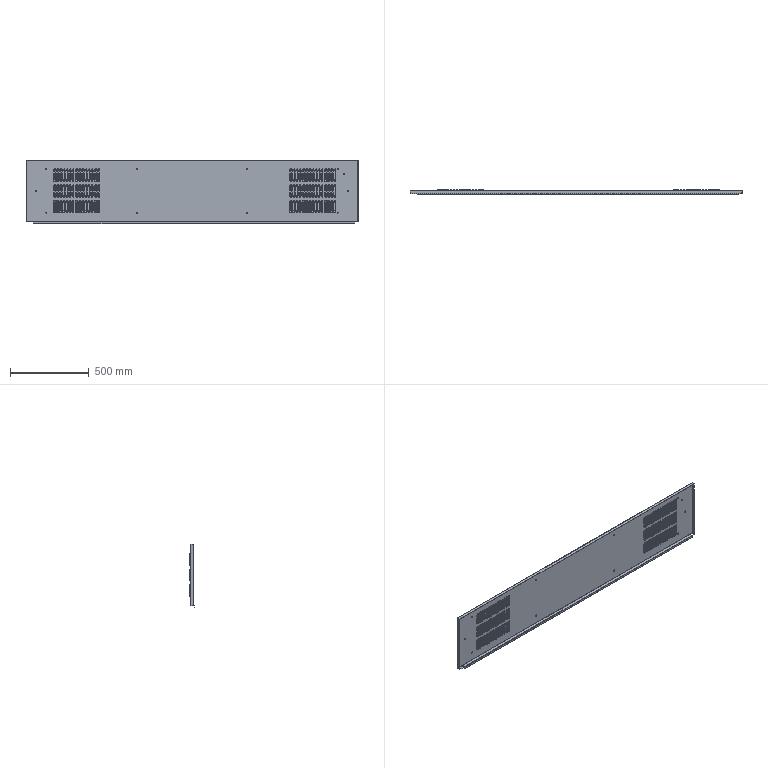Component | SolidWorks | LeftRearDoorAssembly-1_LeftRearDoorWelding-1_LeftRearDoorFrameRiveted-1_LeftRearDoorFramePG50-03-101-1 | 1 solid | 2283 faces | volume 1462240 mm3 | cylinder 1142 | torus 720 | plane 421 | commonest cylinder face diameters 12.38 x270 3.02 x270 15.38 x270 0.02 x270 6 x24 9.3 x22 3.2 x5 0.2 x5